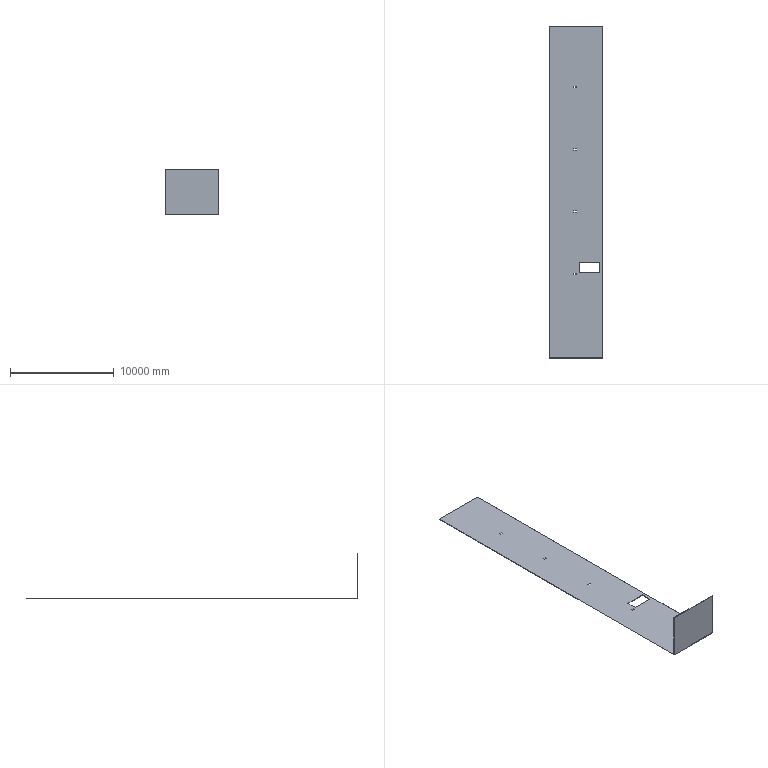Component | SolidWorks | ColorSteelTile-1 | 1 solid | 28 faces | box 5200 x 32004.68 x 4390.02 mm | volume 9342579455 mm3 | plane 28
build123d program:
from build123d import *

# Parameters (mm, degrees)
BOSS_EXTRUDE1_DEPTH       = 5200
CUT_EXTRUDE1_2_DEPTH      = 36550.396
CUT_EXTRUDE1_2_DEPTH_BACK = 36550.396
SKETCH2_W                 = 1000
SKETCH2_H                 = 2000.43
CUT_EXTRUDE1_DEPTH        = 36564.156
CUT_EXTRUDE1_DEPTH_BACK   = 36564.156
SKETCH1_W                 = 135
SKETCH1_H                 = 260


with BuildPart() as part:
    # Sketch1_2 → Boss-Extrude1 (new body)
    with BuildSketch(Plane.XY):
        Polygon((-3905.572, 113.12), (-35910.251, 113.12), (-35910.251, 4503.137), (-35860.251, 4503.137), (-35860.251, 163.12), (-3905.572, 163.12), align=None)
    extrude(amount=BOSS_EXTRUDE1_DEPTH)

    # Sketch2 → Cut-Extrude1_2 (cut, two sides: drawn at the far end of the back side and taken through both)
    with BuildSketch(Plane.XZ.offset(-113.12).offset(-CUT_EXTRUDE1_2_DEPTH_BACK)):
        with Locations((-27185.572, 3893.179)):
            Rectangle(SKETCH2_W, SKETCH2_H)
    extrude(amount=CUT_EXTRUDE1_2_DEPTH + CUT_EXTRUDE1_2_DEPTH_BACK, mode=Mode.SUBTRACT)

    # Sketch1 → Cut-Extrude1 (cut, two sides: drawn at the far end of the back side and taken through both)
    with BuildSketch(Plane(origin=(0, 0, 0), x_dir=(1, 0, 0), z_dir=(0, 1, 0)).offset(-CUT_EXTRUDE1_DEPTH_BACK)):
        with Locations((-9795.572, -2525)):
            Rectangle(SKETCH1_W, SKETCH1_H)
        with Locations((-15795.572, -2525)):
            Rectangle(SKETCH1_W, SKETCH1_H)
        with Locations((-21795.572, -2525)):
            Rectangle(SKETCH1_W, SKETCH1_H)
        with Locations((-27795.572, -2525)):
            Rectangle(SKETCH1_W, SKETCH1_H)
    extrude(amount=CUT_EXTRUDE1_DEPTH + CUT_EXTRUDE1_DEPTH_BACK, mode=Mode.SUBTRACT)


solid = part.part

# Placed as in the assembly
solid = solid.moved(Location((-830.074, 4663.226, -160.714), (90, 90, 0)))
STEP:
#1=CARTESIAN_POINT('',(61.611,-440.939,0.09473));
#2=VERTEX_POINT('',#1);
#3=CARTESIAN_POINT('',(71.847,-440.939,0.09473));
#4=VERTEX_POINT('',#3);
#5=CARTESIAN_POINT('',(1443.87,-440.939,0.09473));
#6=DIRECTION('',(1.,-0.,-0.));
#7=VECTOR('',#6,39.37);
#8=LINE('',#5,#7);
#9=EDGE_CURVE('',#2,#4,#8,.T.);
#10=ORIENTED_EDGE('',*,*,#9,.F.);
#11=CARTESIAN_POINT('',(61.611,-435.624,0.09473));
#12=VERTEX_POINT('',#11);
#13=CARTESIAN_POINT('',(61.611,29.829,0.09473));
#14=DIRECTION('',(-0.,-1.,0.));
#15=VECTOR('',#14,39.37);
#16=LINE('',#13,#15);
#17=EDGE_CURVE('',#12,#2,#16,.T.);
#18=ORIENTED_EDGE('',*,*,#17,.F.);
#19=CARTESIAN_POINT('',(71.847,-435.624,0.09473));
#20=VERTEX_POINT('',#19);
#21=CARTESIAN_POINT('',(1443.87,-435.624,0.09473));
#22=DIRECTION('',(-1.,0.,0.));
#23=VECTOR('',#22,39.37);
#24=LINE('',#21,#23);
#25=EDGE_CURVE('',#20,#12,#24,.T.);
#26=ORIENTED_EDGE('',*,*,#25,.F.);
#27=CARTESIAN_POINT('',(71.847,29.829,0.09473));
#28=DIRECTION('',(0.,1.,-0.));
#29=VECTOR('',#28,39.37);
#30=LINE('',#27,#29);
#31=EDGE_CURVE('',#4,#20,#30,.T.);
#32=ORIENTED_EDGE('',*,*,#31,.F.);
#33=EDGE_LOOP('',(#10,#18,#26,#32));
#34=FACE_BOUND('',#33,.T.);
#35=CARTESIAN_POINT('',(61.611,-913.38,0.09473));
#36=VERTEX_POINT('',#35);
#37=CARTESIAN_POINT('',(71.847,-913.38,0.09473));
#38=VERTEX_POINT('',#37);
#39=CARTESIAN_POINT('',(1443.87,-913.38,0.09473));
#40=DIRECTION('',(1.,-0.,-0.));
#41=VECTOR('',#40,39.37);
#42=LINE('',#39,#41);
#43=EDGE_CURVE('',#36,#38,#42,.T.);
#44=ORIENTED_EDGE('',*,*,#43,.F.);
#45=CARTESIAN_POINT('',(61.611,-908.065,0.09473));
#46=VERTEX_POINT('',#45);
#47=CARTESIAN_POINT('',(61.611,29.829,0.09473));
#48=DIRECTION('',(-0.,-1.,0.));
#49=VECTOR('',#48,39.37);
#50=LINE('',#47,#49);
#51=EDGE_CURVE('',#46,#36,#50,.T.);
#52=ORIENTED_EDGE('',*,*,#51,.F.);
#53=CARTESIAN_POINT('',(71.847,-908.065,0.09473));
#54=VERTEX_POINT('',#53);
#55=CARTESIAN_POINT('',(1443.87,-908.065,0.09473));
#56=DIRECTION('',(-1.,0.,0.));
#57=VECTOR('',#56,39.37);
#58=LINE('',#55,#57);
#59=EDGE_CURVE('',#54,#46,#58,.T.);
#60=ORIENTED_EDGE('',*,*,#59,.F.);
#61=CARTESIAN_POINT('',(71.847,29.829,0.09473));
#62=DIRECTION('',(0.,1.,-0.));
#63=VECTOR('',#62,39.37);
#64=LINE('',#61,#63);
#65=EDGE_CURVE('',#38,#54,#64,.T.);
#66=ORIENTED_EDGE('',*,*,#65,.F.);
#67=EDGE_LOOP('',(#44,#52,#60,#66));
#68=FACE_BOUND('',#67,.T.);
#69=CARTESIAN_POINT('',(159.973,-867.022,0.09473));
#70=VERTEX_POINT('',#69);
#71=CARTESIAN_POINT('',(159.973,-906.392,0.09473));
#72=VERTEX_POINT('',#71);
#73=CARTESIAN_POINT('',(159.973,29.829,0.09473));
#74=DIRECTION('',(0.,-1.,0.));
#75=VECTOR('',#74,39.37);
#76=LINE('',#73,#75);
#77=EDGE_CURVE('',#70,#72,#76,.T.);
#78=ORIENTED_EDGE('',*,*,#77,.T.);
#79=CARTESIAN_POINT('',(81.216,-906.392,0.09473));
#80=VERTEX_POINT('',#79);
#81=CARTESIAN_POINT('',(1443.87,-906.392,0.09473));
#82=DIRECTION('',(-1.,0.,0.));
#83=VECTOR('',#82,39.37);
#84=LINE('',#81,#83);
#85=EDGE_CURVE('',#72,#80,#84,.T.);
#86=ORIENTED_EDGE('',*,*,#85,.T.);
#87=CARTESIAN_POINT('',(81.216,-867.022,0.09473));
#88=VERTEX_POINT('',#87);
#89=CARTESIAN_POINT('',(81.216,29.829,0.09473));
#90=DIRECTION('',(0.,1.,-0.));
#91=VECTOR('',#90,39.37);
#92=LINE('',#89,#91);
#93=EDGE_CURVE('',#80,#88,#92,.T.);
#94=ORIENTED_EDGE('',*,*,#93,.T.);
#95=CARTESIAN_POINT('',(1443.87,-867.022,0.09473));
#96=DIRECTION('',(1.,-0.,-0.));
#97=VECTOR('',#96,39.37);
#98=LINE('',#95,#97);
#99=EDGE_CURVE('',#88,#70,#98,.T.);
#100=ORIENTED_EDGE('',*,*,#99,.T.);
#101=EDGE_LOOP('',(#78,#86,#94,#100));
#102=FACE_BOUND('',#101,.T.);
#103=CARTESIAN_POINT('',(172.044,29.829,0.09473));
#104=VERTEX_POINT('',#103);
#105=CARTESIAN_POINT('',(172.044,-1228.229,0.09473));
#106=VERTEX_POINT('',#105);
#107=CARTESIAN_POINT('',(172.044,29.829,0.09473));
#108=DIRECTION('',(0.,-1.,0.));
#109=VECTOR('',#108,39.37);
#110=LINE('',#107,#109);
#111=EDGE_CURVE('',#104,#106,#110,.T.);
#112=ORIENTED_EDGE('',*,*,#111,.F.);
#113=CARTESIAN_POINT('',(-32.68,29.829,0.09473));
#114=VERTEX_POINT('',#113);
#115=CARTESIAN_POINT('',(1443.87,29.829,0.09473));
#116=DIRECTION('',(-1.,0.,0.));
#117=VECTOR('',#116,39.37);
#118=LINE('',#115,#117);
#119=EDGE_CURVE('',#104,#114,#118,.T.);
#120=ORIENTED_EDGE('',*,*,#119,.T.);
#121=CARTESIAN_POINT('',(-32.68,-1228.229,0.09473));
#122=VERTEX_POINT('',#121);
#123=CARTESIAN_POINT('',(-32.68,29.829,0.09473));
#124=DIRECTION('',(-0.,-1.,0.));
#125=VECTOR('',#124,39.37);
#126=LINE('',#123,#125);
#127=EDGE_CURVE('',#114,#122,#126,.T.);
#128=ORIENTED_EDGE('',*,*,#127,.T.);
#129=CARTESIAN_POINT('',(1443.87,-1228.229,0.09473));
#130=DIRECTION('',(-1.,0.,0.));
#131=VECTOR('',#130,39.37);
#132=LINE('',#129,#131);
#133=EDGE_CURVE('',#106,#122,#132,.T.);
#134=ORIENTED_EDGE('',*,*,#133,.F.);
#135=EDGE_LOOP('',(#112,#120,#128,#134));
#136=FACE_OUTER_BOUND('',#135,.T.);
#137=CARTESIAN_POINT('',(61.611,-677.159,0.09473));
#138=VERTEX_POINT('',#137);
#139=CARTESIAN_POINT('',(71.847,-677.159,0.09473));
#140=VERTEX_POINT('',#139);
#141=CARTESIAN_POINT('',(1443.87,-677.159,0.09473));
#142=DIRECTION('',(1.,-0.,-0.));
#143=VECTOR('',#142,39.37);
#144=LINE('',#141,#143);
#145=EDGE_CURVE('',#138,#140,#144,.T.);
#146=ORIENTED_EDGE('',*,*,#145,.F.);
#147=CARTESIAN_POINT('',(61.611,-671.844,0.09473));
#148=VERTEX_POINT('',#147);
#149=CARTESIAN_POINT('',(61.611,29.829,0.09473));
#150=DIRECTION('',(-0.,-1.,0.));
#151=VECTOR('',#150,39.37);
#152=LINE('',#149,#151);
#153=EDGE_CURVE('',#148,#138,#152,.T.);
#154=ORIENTED_EDGE('',*,*,#153,.F.);
#155=CARTESIAN_POINT('',(71.847,-671.844,0.09473));
#156=VERTEX_POINT('',#155);
#157=CARTESIAN_POINT('',(1443.87,-671.844,0.09473));
#158=DIRECTION('',(-1.,0.,0.));
#159=VECTOR('',#158,39.37);
#160=LINE('',#157,#159);
#161=EDGE_CURVE('',#156,#148,#160,.T.);
#162=ORIENTED_EDGE('',*,*,#161,.F.);
#163=CARTESIAN_POINT('',(71.847,29.829,0.09473));
#164=DIRECTION('',(0.,1.,-0.));
#165=VECTOR('',#164,39.37);
#166=LINE('',#163,#165);
#167=EDGE_CURVE('',#140,#156,#166,.T.);
#168=ORIENTED_EDGE('',*,*,#167,.F.);
#169=EDGE_LOOP('',(#146,#154,#162,#168));
#170=FACE_BOUND('',#169,.T.);
#171=CARTESIAN_POINT('',(61.611,-204.718,0.09473));
#172=VERTEX_POINT('',#171);
#173=CARTESIAN_POINT('',(71.847,-204.718,0.09473));
#174=VERTEX_POINT('',#173);
#175=CARTESIAN_POINT('',(1443.87,-204.718,0.09473));
#176=DIRECTION('',(1.,-0.,-0.));
#177=VECTOR('',#176,39.37);
#178=LINE('',#175,#177);
#179=EDGE_CURVE('',#172,#174,#178,.T.);
#180=ORIENTED_EDGE('',*,*,#179,.F.);
#181=CARTESIAN_POINT('',(61.611,-199.403,0.09473));
#182=VERTEX_POINT('',#181);
#183=CARTESIAN_POINT('',(61.611,29.829,0.09473));
#184=DIRECTION('',(-0.,-1.,0.));
#185=VECTOR('',#184,39.37);
#186=LINE('',#183,#185);
#187=EDGE_CURVE('',#182,#172,#186,.T.);
#188=ORIENTED_EDGE('',*,*,#187,.F.);
#189=CARTESIAN_POINT('',(71.847,-199.403,0.09473));
#190=VERTEX_POINT('',#189);
#191=CARTESIAN_POINT('',(1443.87,-199.403,0.09473));
#192=DIRECTION('',(-1.,0.,0.));
#193=VECTOR('',#192,39.37);
#194=LINE('',#191,#193);
#195=EDGE_CURVE('',#190,#182,#194,.T.);
#196=ORIENTED_EDGE('',*,*,#195,.F.);
#197=CARTESIAN_POINT('',(71.847,29.829,0.09473));
#198=DIRECTION('',(0.,1.,-0.));
#199=VECTOR('',#198,39.37);
#200=LINE('',#197,#199);
#201=EDGE_CURVE('',#174,#190,#200,.T.);
#202=ORIENTED_EDGE('',*,*,#201,.F.);
#203=EDGE_LOOP('',(#180,#188,#196,#202));
#204=FACE_BOUND('',#203,.T.);
#205=CARTESIAN_POINT('',(1443.87,29.829,0.09473));
#206=DIRECTION('',(-0.,-0.,-1.));
#207=DIRECTION('',(-1.,0.,0.));
#208=AXIS2_PLACEMENT_3D('',#205,#206,#207);
#209=PLANE('',#208);
#210=ADVANCED_FACE('',(#34,#68,#102,#136,#170,#204),#209,.F.);
#211=CARTESIAN_POINT('',(71.847,-440.939,-1.874));
#212=VERTEX_POINT('',#211);
#213=CARTESIAN_POINT('',(61.611,-440.939,-1.874));
#214=VERTEX_POINT('',#213);
#215=CARTESIAN_POINT('',(1443.87,-440.939,-1.874));
#216=DIRECTION('',(-1.,0.,0.));
#217=VECTOR('',#216,39.37);
#218=LINE('',#215,#217);
#219=EDGE_CURVE('',#212,#214,#218,.T.);
#220=ORIENTED_EDGE('',*,*,#219,.F.);
#221=CARTESIAN_POINT('',(71.847,-435.624,-1.874));
#222=VERTEX_POINT('',#221);
#223=CARTESIAN_POINT('',(71.847,29.829,-1.874));
#224=DIRECTION('',(-0.,-1.,0.));
#225=VECTOR('',#224,39.37);
#226=LINE('',#223,#225);
#227=EDGE_CURVE('',#222,#212,#226,.T.);
#228=ORIENTED_EDGE('',*,*,#227,.F.);
#229=CARTESIAN_POINT('',(61.611,-435.624,-1.874));
#230=VERTEX_POINT('',#229);
#231=CARTESIAN_POINT('',(1443.87,-435.624,-1.874));
#232=DIRECTION('',(1.,-0.,-0.));
#233=VECTOR('',#232,39.37);
#234=LINE('',#231,#233);
#235=EDGE_CURVE('',#230,#222,#234,.T.);
#236=ORIENTED_EDGE('',*,*,#235,.F.);
#237=CARTESIAN_POINT('',(61.611,29.829,-1.874));
#238=DIRECTION('',(0.,1.,-0.));
#239=VECTOR('',#238,39.37);
#240=LINE('',#237,#239);
#241=EDGE_CURVE('',#214,#230,#240,.T.);
#242=ORIENTED_EDGE('',*,*,#241,.F.);
#243=EDGE_LOOP('',(#220,#228,#236,#242));
#244=FACE_BOUND('',#243,.T.);
#245=CARTESIAN_POINT('',(71.847,-913.38,-1.874));
#246=VERTEX_POINT('',#245);
#247=CARTESIAN_POINT('',(61.611,-913.38,-1.874));
#248=VERTEX_POINT('',#247);
#249=CARTESIAN_POINT('',(1443.87,-913.38,-1.874));
#250=DIRECTION('',(-1.,0.,0.));
#251=VECTOR('',#250,39.37);
#252=LINE('',#249,#251);
#253=EDGE_CURVE('',#246,#248,#252,.T.);
#254=ORIENTED_EDGE('',*,*,#253,.F.);
#255=CARTESIAN_POINT('',(71.847,-908.065,-1.874));
#256=VERTEX_POINT('',#255);
#257=CARTESIAN_POINT('',(71.847,29.829,-1.874));
#258=DIRECTION('',(-0.,-1.,0.));
#259=VECTOR('',#258,39.37);
#260=LINE('',#257,#259);
#261=EDGE_CURVE('',#256,#246,#260,.T.);
#262=ORIENTED_EDGE('',*,*,#261,.F.);
#263=CARTESIAN_POINT('',(61.611,-908.065,-1.874));
#264=VERTEX_POINT('',#263);
#265=CARTESIAN_POINT('',(1443.87,-908.065,-1.874));
#266=DIRECTION('',(1.,-0.,-0.));
#267=VECTOR('',#266,39.37);
#268=LINE('',#265,#267);
#269=EDGE_CURVE('',#264,#256,#268,.T.);
#270=ORIENTED_EDGE('',*,*,#269,.F.);
#271=CARTESIAN_POINT('',(61.611,29.829,-1.874));
#272=DIRECTION('',(0.,1.,-0.));
#273=VECTOR('',#272,39.37);
#274=LINE('',#271,#273);
#275=EDGE_CURVE('',#248,#264,#274,.T.);
#276=ORIENTED_EDGE('',*,*,#275,.F.);
#277=EDGE_LOOP('',(#254,#262,#270,#276));
#278=FACE_BOUND('',#277,.T.);
#279=CARTESIAN_POINT('',(81.216,-867.022,-1.874));
#280=VERTEX_POINT('',#279);
#281=CARTESIAN_POINT('',(81.216,-906.392,-1.874));
#282=VERTEX_POINT('',#281);
#283=CARTESIAN_POINT('',(81.216,29.829,-1.874));
#284=DIRECTION('',(-0.,-1.,0.));
#285=VECTOR('',#284,39.37);
#286=LINE('',#283,#285);
#287=EDGE_CURVE('',#280,#282,#286,.T.);
#288=ORIENTED_EDGE('',*,*,#287,.T.);
#289=CARTESIAN_POINT('',(159.973,-906.392,-1.874));
#290=VERTEX_POINT('',#289);
#291=CARTESIAN_POINT('',(1443.87,-906.392,-1.874));
#292=DIRECTION('',(1.,-0.,-0.));
#293=VECTOR('',#292,39.37);
#294=LINE('',#291,#293);
#295=EDGE_CURVE('',#282,#290,#294,.T.);
#296=ORIENTED_EDGE('',*,*,#295,.T.);
#297=CARTESIAN_POINT('',(159.973,-867.022,-1.874));
#298=VERTEX_POINT('',#297);
#299=CARTESIAN_POINT('',(159.973,29.829,-1.874));
#300=DIRECTION('',(-0.,1.,-0.));
#301=VECTOR('',#300,39.37);
#302=LINE('',#299,#301);
#303=EDGE_CURVE('',#290,#298,#302,.T.);
#304=ORIENTED_EDGE('',*,*,#303,.T.);
#305=CARTESIAN_POINT('',(1443.87,-867.022,-1.874));
#306=DIRECTION('',(-1.,0.,0.));
#307=VECTOR('',#306,39.37);
#308=LINE('',#305,#307);
#309=EDGE_CURVE('',#298,#280,#308,.T.);
#310=ORIENTED_EDGE('',*,*,#309,.T.);
#311=EDGE_LOOP('',(#288,#296,#304,#310));
#312=FACE_BOUND('',#311,.T.);
#313=CARTESIAN_POINT('',(172.044,-1230.198,-1.874));
#314=VERTEX_POINT('',#313);
#315=CARTESIAN_POINT('',(172.044,29.829,-1.874));
#316=VERTEX_POINT('',#315);
#317=CARTESIAN_POINT('',(172.044,29.829,-1.874));
#318=DIRECTION('',(0.,1.,-0.));
#319=VECTOR('',#318,39.37);
#320=LINE('',#317,#319);
#321=EDGE_CURVE('',#314,#316,#320,.T.);
#322=ORIENTED_EDGE('',*,*,#321,.F.);
#323=CARTESIAN_POINT('',(-32.68,-1230.198,-1.874));
#324=VERTEX_POINT('',#323);
#325=CARTESIAN_POINT('',(1443.87,-1230.198,-1.874));
#326=DIRECTION('',(-1.,0.,0.));
#327=VECTOR('',#326,39.37);
#328=LINE('',#325,#327);
#329=EDGE_CURVE('',#314,#324,#328,.T.);
#330=ORIENTED_EDGE('',*,*,#329,.T.);
#331=CARTESIAN_POINT('',(-32.68,29.829,-1.874));
#332=VERTEX_POINT('',#331);
#333=CARTESIAN_POINT('',(-32.68,29.829,-1.874));
#334=DIRECTION('',(0.,1.,-0.));
#335=VECTOR('',#334,39.37);
#336=LINE('',#333,#335);
#337=EDGE_CURVE('',#324,#332,#336,.T.);
#338=ORIENTED_EDGE('',*,*,#337,.T.);
#339=CARTESIAN_POINT('',(1443.87,29.829,-1.874));
#340=DIRECTION('',(-1.,0.,0.));
#341=VECTOR('',#340,39.37);
#342=LINE('',#339,#341);
#343=EDGE_CURVE('',#316,#332,#342,.T.);
#344=ORIENTED_EDGE('',*,*,#343,.F.);
#345=EDGE_LOOP('',(#322,#330,#338,#344));
#346=FACE_OUTER_BOUND('',#345,.T.);
#347=CARTESIAN_POINT('',(71.847,-677.159,-1.874));
#348=VERTEX_POINT('',#347);
#349=CARTESIAN_POINT('',(61.611,-677.159,-1.874));
#350=VERTEX_POINT('',#349);
#351=CARTESIAN_POINT('',(1443.87,-677.159,-1.874));
#352=DIRECTION('',(-1.,0.,0.));
#353=VECTOR('',#352,39.37);
#354=LINE('',#351,#353);
#355=EDGE_CURVE('',#348,#350,#354,.T.);
#356=ORIENTED_EDGE('',*,*,#355,.F.);
#357=CARTESIAN_POINT('',(71.847,-671.844,-1.874));
#358=VERTEX_POINT('',#357);
#359=CARTESIAN_POINT('',(71.847,29.829,-1.874));
#360=DIRECTION('',(-0.,-1.,0.));
#361=VECTOR('',#360,39.37);
#362=LINE('',#359,#361);
#363=EDGE_CURVE('',#358,#348,#362,.T.);
#364=ORIENTED_EDGE('',*,*,#363,.F.);
#365=CARTESIAN_POINT('',(61.611,-671.844,-1.874));
#366=VERTEX_POINT('',#365);
#367=CARTESIAN_POINT('',(1443.87,-671.844,-1.874));
#368=DIRECTION('',(1.,-0.,-0.));
#369=VECTOR('',#368,39.37);
#370=LINE('',#367,#369);
#371=EDGE_CURVE('',#366,#358,#370,.T.);
#372=ORIENTED_EDGE('',*,*,#371,.F.);
#373=CARTESIAN_POINT('',(61.611,29.829,-1.874));
#374=DIRECTION('',(0.,1.,-0.));
#375=VECTOR('',#374,39.37);
#376=LINE('',#373,#375);
#377=EDGE_CURVE('',#350,#366,#376,.T.);
#378=ORIENTED_EDGE('',*,*,#377,.F.);
#379=EDGE_LOOP('',(#356,#364,#372,#378));
#380=FACE_BOUND('',#379,.T.);
#381=CARTESIAN_POINT('',(71.847,-204.718,-1.874));
#382=VERTEX_POINT('',#381);
#383=CARTESIAN_POINT('',(61.611,-204.718,-1.874));
#384=VERTEX_POINT('',#383);
#385=CARTESIAN_POINT('',(1443.87,-204.718,-1.874));
#386=DIRECTION('',(-1.,0.,0.));
#387=VECTOR('',#386,39.37);
#388=LINE('',#385,#387);
#389=EDGE_CURVE('',#382,#384,#388,.T.);
#390=ORIENTED_EDGE('',*,*,#389,.F.);
#391=CARTESIAN_POINT('',(71.847,-199.403,-1.874));
#392=VERTEX_POINT('',#391);
#393=CARTESIAN_POINT('',(71.847,29.829,-1.874));
#394=DIRECTION('',(-0.,-1.,0.));
#395=VECTOR('',#394,39.37);
#396=LINE('',#393,#395);
#397=EDGE_CURVE('',#392,#382,#396,.T.);
#398=ORIENTED_EDGE('',*,*,#397,.F.);
#399=CARTESIAN_POINT('',(61.611,-199.403,-1.874));
#400=VERTEX_POINT('',#399);
#401=CARTESIAN_POINT('',(1443.87,-199.403,-1.874));
#402=DIRECTION('',(1.,-0.,-0.));
#403=VECTOR('',#402,39.37);
#404=LINE('',#401,#403);
#405=EDGE_CURVE('',#400,#392,#404,.T.);
#406=ORIENTED_EDGE('',*,*,#405,.F.);
#407=CARTESIAN_POINT('',(61.611,29.829,-1.874));
#408=DIRECTION('',(0.,1.,-0.));
#409=VECTOR('',#408,39.37);
#410=LINE('',#407,#409);
#411=EDGE_CURVE('',#384,#400,#410,.T.);
#412=ORIENTED_EDGE('',*,*,#411,.F.);
#413=EDGE_LOOP('',(#390,#398,#406,#412));
#414=FACE_BOUND('',#413,.T.);
#415=CARTESIAN_POINT('',(1443.87,29.829,-1.874));
#416=DIRECTION('',(0.,0.,1.));
#417=DIRECTION('',(1.,-0.,-0.));
#418=AXIS2_PLACEMENT_3D('',#415,#416,#417);
#419=PLANE('',#418);
#420=ADVANCED_FACE('',(#244,#278,#312,#346,#380,#414),#419,.F.);
#421=CARTESIAN_POINT('',(172.044,29.829,-1.874));
#422=DIRECTION('',(0.,0.,1.));
#423=VECTOR('',#422,39.37);
#424=LINE('',#421,#423);
#425=EDGE_CURVE('',#316,#104,#424,.T.);
#426=ORIENTED_EDGE('',*,*,#425,.F.);
#427=ORIENTED_EDGE('',*,*,#343,.T.);
#428=CARTESIAN_POINT('',(-32.68,29.829,-1.874));
#429=DIRECTION('',(0.,0.,1.));
#430=VECTOR('',#429,39.37);
#431=LINE('',#428,#430);
#432=EDGE_CURVE('',#332,#114,#431,.T.);
#433=ORIENTED_EDGE('',*,*,#432,.T.);
#434=ORIENTED_EDGE('',*,*,#119,.F.);
#435=EDGE_LOOP('',(#426,#427,#433,#434));
#436=FACE_OUTER_BOUND('',#435,.T.);
#437=CARTESIAN_POINT('',(1443.87,29.829,-1.874));
#438=DIRECTION('',(-0.,-1.,0.));
#439=DIRECTION('',(1.,-0.,-0.));
#440=AXIS2_PLACEMENT_3D('',#437,#438,#439);
#441=PLANE('',#440);
#442=ADVANCED_FACE('',(#436),#441,.F.);
#443=CARTESIAN_POINT('',(172.044,-1228.229,170.962));
#444=VERTEX_POINT('',#443);
#445=CARTESIAN_POINT('',(172.044,-1228.229,0.09473));
#446=DIRECTION('',(0.,0.,1.));
#447=VECTOR('',#446,39.37);
#448=LINE('',#445,#447);
#449=EDGE_CURVE('',#106,#444,#448,.T.);
#450=ORIENTED_EDGE('',*,*,#449,.F.);
#451=ORIENTED_EDGE('',*,*,#133,.T.);
#452=CARTESIAN_POINT('',(-32.68,-1228.229,170.962));
#453=VERTEX_POINT('',#452);
#454=CARTESIAN_POINT('',(-32.68,-1228.229,0.09473));
#455=DIRECTION('',(0.,0.,1.));
#456=VECTOR('',#455,39.37);
#457=LINE('',#454,#456);
#458=EDGE_CURVE('',#122,#453,#457,.T.);
#459=ORIENTED_EDGE('',*,*,#458,.T.);
#460=CARTESIAN_POINT('',(1443.87,-1228.229,170.962));
#461=DIRECTION('',(-1.,0.,0.));
#462=VECTOR('',#461,39.37);
#463=LINE('',#460,#462);
#464=EDGE_CURVE('',#444,#453,#463,.T.);
#465=ORIENTED_EDGE('',*,*,#464,.F.);
#466=EDGE_LOOP('',(#450,#451,#459,#465));
#467=FACE_OUTER_BOUND('',#466,.T.);
#468=CARTESIAN_POINT('',(1443.87,-1228.229,0.09473));
#469=DIRECTION('',(-0.,-1.,0.));
#470=DIRECTION('',(1.,-0.,-0.));
#471=AXIS2_PLACEMENT_3D('',#468,#469,#470);
#472=PLANE('',#471);
#473=ADVANCED_FACE('',(#467),#472,.F.);
#474=CARTESIAN_POINT('',(172.044,-1230.198,170.962));
#475=VERTEX_POINT('',#474);
#476=CARTESIAN_POINT('',(172.044,-1228.229,170.962));
#477=DIRECTION('',(0.,-1.,0.));
#478=VECTOR('',#477,39.37);
#479=LINE('',#476,#478);
#480=EDGE_CURVE('',#444,#475,#479,.T.);
#481=ORIENTED_EDGE('',*,*,#480,.F.);
#482=ORIENTED_EDGE('',*,*,#464,.T.);
#483=CARTESIAN_POINT('',(-32.68,-1230.198,170.962));
#484=VERTEX_POINT('',#483);
#485=CARTESIAN_POINT('',(-32.68,-1228.229,170.962));
#486=DIRECTION('',(-0.,-1.,0.));
#487=VECTOR('',#486,39.37);
#488=LINE('',#485,#487);
#489=EDGE_CURVE('',#453,#484,#488,.T.);
#490=ORIENTED_EDGE('',*,*,#489,.T.);
#491=CARTESIAN_POINT('',(1443.87,-1230.198,170.962));
#492=DIRECTION('',(-1.,0.,0.));
#493=VECTOR('',#492,39.37);
#494=LINE('',#491,#493);
#495=EDGE_CURVE('',#475,#484,#494,.T.);
#496=ORIENTED_EDGE('',*,*,#495,.F.);
#497=EDGE_LOOP('',(#481,#482,#490,#496));
#498=FACE_OUTER_BOUND('',#497,.T.);
#499=CARTESIAN_POINT('',(1443.87,-1228.229,170.962));
#500=DIRECTION('',(-0.,-0.,-1.));
#501=DIRECTION('',(-1.,0.,0.));
#502=AXIS2_PLACEMENT_3D('',#499,#500,#501);
#503=PLANE('',#502);
#504=ADVANCED_FACE('',(#498),#503,.F.);
#505=CARTESIAN_POINT('',(172.044,-1230.198,-1.874));
#506=DIRECTION('',(0.,-0.,-1.));
#507=VECTOR('',#506,39.37);
#508=LINE('',#505,#507);
#509=EDGE_CURVE('',#475,#314,#508,.T.);
#510=ORIENTED_EDGE('',*,*,#509,.F.);
#511=ORIENTED_EDGE('',*,*,#495,.T.);
#512=CARTESIAN_POINT('',(-32.68,-1230.198,-1.874));
#513=DIRECTION('',(-0.,-0.,-1.));
#514=VECTOR('',#513,39.37);
#515=LINE('',#512,#514);
#516=EDGE_CURVE('',#484,#324,#515,.T.);
#517=ORIENTED_EDGE('',*,*,#516,.T.);
#518=ORIENTED_EDGE('',*,*,#329,.F.);
#519=EDGE_LOOP('',(#510,#511,#517,#518));
#520=FACE_OUTER_BOUND('',#519,.T.);
#521=CARTESIAN_POINT('',(1443.87,-1230.198,-1.874));
#522=DIRECTION('',(0.,1.,-0.));
#523=DIRECTION('',(-1.,0.,0.));
#524=AXIS2_PLACEMENT_3D('',#521,#522,#523);
#525=PLANE('',#524);
#526=ADVANCED_FACE('',(#520),#525,.F.);
#527=ORIENTED_EDGE('',*,*,#432,.F.);
#528=ORIENTED_EDGE('',*,*,#337,.F.);
#529=ORIENTED_EDGE('',*,*,#516,.F.);
#530=ORIENTED_EDGE('',*,*,#489,.F.);
#531=ORIENTED_EDGE('',*,*,#458,.F.);
#532=ORIENTED_EDGE('',*,*,#127,.F.);
#533=EDGE_LOOP('',(#527,#528,#529,#530,#531,#532));
#534=FACE_OUTER_BOUND('',#533,.T.);
#535=CARTESIAN_POINT('',(-32.68,183.592,-6.327));
#536=DIRECTION('',(1.,-0.,-0.));
#537=DIRECTION('',(0.,1.,-0.));
#538=AXIS2_PLACEMENT_3D('',#535,#536,#537);
#539=PLANE('',#538);
#540=ADVANCED_FACE('',(#534),#539,.F.);
#541=ORIENTED_EDGE('',*,*,#321,.T.);
#542=ORIENTED_EDGE('',*,*,#425,.T.);
#543=ORIENTED_EDGE('',*,*,#111,.T.);
#544=ORIENTED_EDGE('',*,*,#449,.T.);
#545=ORIENTED_EDGE('',*,*,#480,.T.);
#546=ORIENTED_EDGE('',*,*,#509,.T.);
#547=EDGE_LOOP('',(#541,#542,#543,#544,#545,#546));
#548=FACE_OUTER_BOUND('',#547,.T.);
#549=CARTESIAN_POINT('',(172.044,-705.073,-17.704));
#550=DIRECTION('',(1.,0.,-0.));
#551=DIRECTION('',(0.,-0.,-1.));
#552=AXIS2_PLACEMENT_3D('',#549,#550,#551);
#553=PLANE('',#552);
#554=ADVANCED_FACE('',(#548),#553,.T.);
#555=CARTESIAN_POINT('',(159.973,-906.392,170.962));
#556=DIRECTION('',(-0.,0.,-1.));
#557=VECTOR('',#556,39.37);
#558=LINE('',#555,#557);
#559=EDGE_CURVE('',#72,#290,#558,.T.);
#560=ORIENTED_EDGE('',*,*,#559,.T.);
#561=ORIENTED_EDGE('',*,*,#295,.F.);
#562=CARTESIAN_POINT('',(81.216,-906.392,170.962));
#563=DIRECTION('',(-0.,0.,-1.));
#564=VECTOR('',#563,39.37);
#565=LINE('',#562,#564);
#566=EDGE_CURVE('',#80,#282,#565,.T.);
#567=ORIENTED_EDGE('',*,*,#566,.F.);
#568=ORIENTED_EDGE('',*,*,#85,.F.);
#569=EDGE_LOOP('',(#560,#561,#567,#568));
#570=FACE_OUTER_BOUND('',#569,.T.);
#571=CARTESIAN_POINT('',(159.973,-906.392,170.962));
#572=DIRECTION('',(-0.,-1.,-0.));
#573=DIRECTION('',(-0.,0.,-1.));
#574=AXIS2_PLACEMENT_3D('',#571,#572,#573);
#575=PLANE('',#574);
#576=ADVANCED_FACE('',(#570),#575,.F.);
#577=CARTESIAN_POINT('',(159.973,-867.022,170.962));
#578=DIRECTION('',(-0.,0.,-1.));
#579=VECTOR('',#578,39.37);
#580=LINE('',#577,#579);
#581=EDGE_CURVE('',#70,#298,#580,.T.);
#582=ORIENTED_EDGE('',*,*,#581,.T.);
#583=ORIENTED_EDGE('',*,*,#303,.F.);
#584=ORIENTED_EDGE('',*,*,#559,.F.);
#585=ORIENTED_EDGE('',*,*,#77,.F.);
#586=EDGE_LOOP('',(#582,#583,#584,#585));
#587=FACE_OUTER_BOUND('',#586,.T.);
#588=CARTESIAN_POINT('',(159.973,-906.392,170.962));
#589=DIRECTION('',(1.,0.,-0.));
#590=DIRECTION('',(-0.,1.,-0.));
#591=AXIS2_PLACEMENT_3D('',#588,#589,#590);
#592=PLANE('',#591);
#593=ADVANCED_FACE('',(#587),#592,.F.);
#594=CARTESIAN_POINT('',(81.216,-867.022,170.962));
#595=DIRECTION('',(-0.,0.,-1.));
#596=VECTOR('',#595,39.37);
#597=LINE('',#594,#596);
#598=EDGE_CURVE('',#88,#280,#597,.T.);
#599=ORIENTED_EDGE('',*,*,#598,.T.);
#600=ORIENTED_EDGE('',*,*,#309,.F.);
#601=ORIENTED_EDGE('',*,*,#581,.F.);
#602=ORIENTED_EDGE('',*,*,#99,.F.);
#603=EDGE_LOOP('',(#599,#600,#601,#602));
#604=FACE_OUTER_BOUND('',#603,.T.);
#605=CARTESIAN_POINT('',(159.973,-867.022,170.962));
#606=DIRECTION('',(0.,1.,0.));
#607=DIRECTION('',(0.,-0.,1.));
#608=AXIS2_PLACEMENT_3D('',#605,#606,#607);
#609=PLANE('',#608);
#610=ADVANCED_FACE('',(#604),#609,.F.);
#611=ORIENTED_EDGE('',*,*,#566,.T.);
#612=ORIENTED_EDGE('',*,*,#287,.F.);
#613=ORIENTED_EDGE('',*,*,#598,.F.);
#614=ORIENTED_EDGE('',*,*,#93,.F.);
#615=EDGE_LOOP('',(#611,#612,#613,#614));
#616=FACE_OUTER_BOUND('',#615,.T.);
#617=CARTESIAN_POINT('',(81.216,-906.392,170.962));
#618=DIRECTION('',(-1.,0.,0.));
#619=DIRECTION('',(-0.,-1.,0.));
#620=AXIS2_PLACEMENT_3D('',#617,#618,#619);
#621=PLANE('',#620);
#622=ADVANCED_FACE('',(#616),#621,.F.);
#623=ORIENTED_EDGE('',*,*,#43,.T.);
#624=CARTESIAN_POINT('',(71.847,-913.38,-1.874));
#625=DIRECTION('',(-0.,-0.,-1.));
#626=VECTOR('',#625,39.37);
#627=LINE('',#624,#626);
#628=EDGE_CURVE('',#38,#246,#627,.T.);
#629=ORIENTED_EDGE('',*,*,#628,.T.);
#630=ORIENTED_EDGE('',*,*,#253,.T.);
#631=CARTESIAN_POINT('',(61.611,-913.38,-1.874));
#632=DIRECTION('',(-0.,-0.,-1.));
#633=VECTOR('',#632,39.37);
#634=LINE('',#631,#633);
#635=EDGE_CURVE('',#36,#248,#634,.T.);
#636=ORIENTED_EDGE('',*,*,#635,.F.);
#637=EDGE_LOOP('',(#623,#629,#630,#636));
#638=FACE_OUTER_BOUND('',#637,.T.);
#639=CARTESIAN_POINT('',(61.611,-913.38,-1.874));
#640=DIRECTION('',(0.,1.,-0.));
#641=DIRECTION('',(-1.,0.,0.));
#642=AXIS2_PLACEMENT_3D('',#639,#640,#641);
#643=PLANE('',#642);
#644=ADVANCED_FACE('',(#638),#643,.T.);
#645=ORIENTED_EDGE('',*,*,#65,.T.);
#646=CARTESIAN_POINT('',(71.847,-908.065,-1.874));
#647=DIRECTION('',(-0.,-0.,-1.));
#648=VECTOR('',#647,39.37);
#649=LINE('',#646,#648);
#650=EDGE_CURVE('',#54,#256,#649,.T.);
#651=ORIENTED_EDGE('',*,*,#650,.T.);
#652=ORIENTED_EDGE('',*,*,#261,.T.);
#653=ORIENTED_EDGE('',*,*,#628,.F.);
#654=EDGE_LOOP('',(#645,#651,#652,#653));
#655=FACE_OUTER_BOUND('',#654,.T.);
#656=CARTESIAN_POINT('',(71.847,-913.38,-1.874));
#657=DIRECTION('',(-1.,0.,0.));
#658=DIRECTION('',(-0.,-1.,0.));
#659=AXIS2_PLACEMENT_3D('',#656,#657,#658);
#660=PLANE('',#659);
#661=ADVANCED_FACE('',(#655),#660,.T.);
#662=ORIENTED_EDGE('',*,*,#59,.T.);
#663=CARTESIAN_POINT('',(61.611,-908.065,-1.874));
#664=DIRECTION('',(-0.,-0.,-1.));
#665=VECTOR('',#664,39.37);
#666=LINE('',#663,#665);
#667=EDGE_CURVE('',#46,#264,#666,.T.);
#668=ORIENTED_EDGE('',*,*,#667,.T.);
#669=ORIENTED_EDGE('',*,*,#269,.T.);
#670=ORIENTED_EDGE('',*,*,#650,.F.);
#671=EDGE_LOOP('',(#662,#668,#669,#670));
#672=FACE_OUTER_BOUND('',#671,.T.);
#673=CARTESIAN_POINT('',(61.611,-908.065,-1.874));
#674=DIRECTION('',(-0.,-1.,0.));
#675=DIRECTION('',(1.,-0.,-0.));
#676=AXIS2_PLACEMENT_3D('',#673,#674,#675);
#677=PLANE('',#676);
#678=ADVANCED_FACE('',(#672),#677,.T.);
#679=ORIENTED_EDGE('',*,*,#51,.T.);
#680=ORIENTED_EDGE('',*,*,#635,.T.);
#681=ORIENTED_EDGE('',*,*,#275,.T.);
#682=ORIENTED_EDGE('',*,*,#667,.F.);
#683=EDGE_LOOP('',(#679,#680,#681,#682));
#684=FACE_OUTER_BOUND('',#683,.T.);
#685=CARTESIAN_POINT('',(61.611,-913.38,-1.874));
#686=DIRECTION('',(1.,-0.,-0.));
#687=DIRECTION('',(0.,1.,-0.));
#688=AXIS2_PLACEMENT_3D('',#685,#686,#687);
#689=PLANE('',#688);
#690=ADVANCED_FACE('',(#684),#689,.T.);
#691=ORIENTED_EDGE('',*,*,#145,.T.);
#692=CARTESIAN_POINT('',(71.847,-677.159,-1.874));
#693=DIRECTION('',(-0.,-0.,-1.));
#694=VECTOR('',#693,39.37);
#695=LINE('',#692,#694);
#696=EDGE_CURVE('',#140,#348,#695,.T.);
#697=ORIENTED_EDGE('',*,*,#696,.T.);
#698=ORIENTED_EDGE('',*,*,#355,.T.);
#699=CARTESIAN_POINT('',(61.611,-677.159,-1.874));
#700=DIRECTION('',(-0.,-0.,-1.));
#701=VECTOR('',#700,39.37);
#702=LINE('',#699,#701);
#703=EDGE_CURVE('',#138,#350,#702,.T.);
#704=ORIENTED_EDGE('',*,*,#703,.F.);
#705=EDGE_LOOP('',(#691,#697,#698,#704));
#706=FACE_OUTER_BOUND('',#705,.T.);
#707=CARTESIAN_POINT('',(61.611,-677.159,-1.874));
#708=DIRECTION('',(0.,1.,-0.));
#709=DIRECTION('',(-1.,0.,0.));
#710=AXIS2_PLACEMENT_3D('',#707,#708,#709);
#711=PLANE('',#710);
#712=ADVANCED_FACE('',(#706),#711,.T.);
#713=ORIENTED_EDGE('',*,*,#167,.T.);
#714=CARTESIAN_POINT('',(71.847,-671.844,-1.874));
#715=DIRECTION('',(-0.,-0.,-1.));
#716=VECTOR('',#715,39.37);
#717=LINE('',#714,#716);
#718=EDGE_CURVE('',#156,#358,#717,.T.);
#719=ORIENTED_EDGE('',*,*,#718,.T.);
#720=ORIENTED_EDGE('',*,*,#363,.T.);
#721=ORIENTED_EDGE('',*,*,#696,.F.);
#722=EDGE_LOOP('',(#713,#719,#720,#721));
#723=FACE_OUTER_BOUND('',#722,.T.);
#724=CARTESIAN_POINT('',(71.847,-677.159,-1.874));
#725=DIRECTION('',(-1.,0.,0.));
#726=DIRECTION('',(-0.,-1.,0.));
#727=AXIS2_PLACEMENT_3D('',#724,#725,#726);
#728=PLANE('',#727);
#729=ADVANCED_FACE('',(#723),#728,.T.);
#730=ORIENTED_EDGE('',*,*,#161,.T.);
#731=CARTESIAN_POINT('',(61.611,-671.844,-1.874));
#732=DIRECTION('',(-0.,-0.,-1.));
#733=VECTOR('',#732,39.37);
#734=LINE('',#731,#733);
#735=EDGE_CURVE('',#148,#366,#734,.T.);
#736=ORIENTED_EDGE('',*,*,#735,.T.);
#737=ORIENTED_EDGE('',*,*,#371,.T.);
#738=ORIENTED_EDGE('',*,*,#718,.F.);
#739=EDGE_LOOP('',(#730,#736,#737,#738));
#740=FACE_OUTER_BOUND('',#739,.T.);
#741=CARTESIAN_POINT('',(61.611,-671.844,-1.874));
#742=DIRECTION('',(-0.,-1.,0.));
#743=DIRECTION('',(1.,-0.,-0.));
#744=AXIS2_PLACEMENT_3D('',#741,#742,#743);
#745=PLANE('',#744);
#746=ADVANCED_FACE('',(#740),#745,.T.);
#747=ORIENTED_EDGE('',*,*,#153,.T.);
#748=ORIENTED_EDGE('',*,*,#703,.T.);
#749=ORIENTED_EDGE('',*,*,#377,.T.);
#750=ORIENTED_EDGE('',*,*,#735,.F.);
#751=EDGE_LOOP('',(#747,#748,#749,#750));
#752=FACE_OUTER_BOUND('',#751,.T.);
#753=CARTESIAN_POINT('',(61.611,-677.159,-1.874));
#754=DIRECTION('',(1.,-0.,-0.));
#755=DIRECTION('',(0.,1.,-0.));
#756=AXIS2_PLACEMENT_3D('',#753,#754,#755);
#757=PLANE('',#756);
#758=ADVANCED_FACE('',(#752),#757,.T.);
#759=ORIENTED_EDGE('',*,*,#9,.T.);
#760=CARTESIAN_POINT('',(71.847,-440.939,-1.874));
#761=DIRECTION('',(-0.,-0.,-1.));
#762=VECTOR('',#761,39.37);
#763=LINE('',#760,#762);
#764=EDGE_CURVE('',#4,#212,#763,.T.);
#765=ORIENTED_EDGE('',*,*,#764,.T.);
#766=ORIENTED_EDGE('',*,*,#219,.T.);
#767=CARTESIAN_POINT('',(61.611,-440.939,-1.874));
#768=DIRECTION('',(-0.,-0.,-1.));
#769=VECTOR('',#768,39.37);
#770=LINE('',#767,#769);
#771=EDGE_CURVE('',#2,#214,#770,.T.);
#772=ORIENTED_EDGE('',*,*,#771,.F.);
#773=EDGE_LOOP('',(#759,#765,#766,#772));
#774=FACE_OUTER_BOUND('',#773,.T.);
#775=CARTESIAN_POINT('',(61.611,-440.939,-1.874));
#776=DIRECTION('',(0.,1.,-0.));
#777=DIRECTION('',(-1.,0.,0.));
#778=AXIS2_PLACEMENT_3D('',#775,#776,#777);
#779=PLANE('',#778);
#780=ADVANCED_FACE('',(#774),#779,.T.);
#781=ORIENTED_EDGE('',*,*,#31,.T.);
#782=CARTESIAN_POINT('',(71.847,-435.624,-1.874));
#783=DIRECTION('',(-0.,-0.,-1.));
#784=VECTOR('',#783,39.37);
#785=LINE('',#782,#784);
#786=EDGE_CURVE('',#20,#222,#785,.T.);
#787=ORIENTED_EDGE('',*,*,#786,.T.);
#788=ORIENTED_EDGE('',*,*,#227,.T.);
#789=ORIENTED_EDGE('',*,*,#764,.F.);
#790=EDGE_LOOP('',(#781,#787,#788,#789));
#791=FACE_OUTER_BOUND('',#790,.T.);
#792=CARTESIAN_POINT('',(71.847,-440.939,-1.874));
#793=DIRECTION('',(-1.,0.,0.));
#794=DIRECTION('',(-0.,-1.,0.));
#795=AXIS2_PLACEMENT_3D('',#792,#793,#794);
#796=PLANE('',#795);
#797=ADVANCED_FACE('',(#791),#796,.T.);
#798=ORIENTED_EDGE('',*,*,#25,.T.);
#799=CARTESIAN_POINT('',(61.611,-435.624,-1.874));
#800=DIRECTION('',(-0.,-0.,-1.));
#801=VECTOR('',#800,39.37);
#802=LINE('',#799,#801);
#803=EDGE_CURVE('',#12,#230,#802,.T.);
#804=ORIENTED_EDGE('',*,*,#803,.T.);
#805=ORIENTED_EDGE('',*,*,#235,.T.);
#806=ORIENTED_EDGE('',*,*,#786,.F.);
#807=EDGE_LOOP('',(#798,#804,#805,#806));
#808=FACE_OUTER_BOUND('',#807,.T.);
#809=CARTESIAN_POINT('',(61.611,-435.624,-1.874));
#810=DIRECTION('',(-0.,-1.,0.));
#811=DIRECTION('',(1.,-0.,-0.));
#812=AXIS2_PLACEMENT_3D('',#809,#810,#811);
#813=PLANE('',#812);
#814=ADVANCED_FACE('',(#808),#813,.T.);
#815=ORIENTED_EDGE('',*,*,#17,.T.);
#816=ORIENTED_EDGE('',*,*,#771,.T.);
#817=ORIENTED_EDGE('',*,*,#241,.T.);
#818=ORIENTED_EDGE('',*,*,#803,.F.);
#819=EDGE_LOOP('',(#815,#816,#817,#818));
#820=FACE_OUTER_BOUND('',#819,.T.);
#821=CARTESIAN_POINT('',(61.611,-440.939,-1.874));
#822=DIRECTION('',(1.,-0.,-0.));
#823=DIRECTION('',(0.,1.,-0.));
#824=AXIS2_PLACEMENT_3D('',#821,#822,#823);
#825=PLANE('',#824);
#826=ADVANCED_FACE('',(#820),#825,.T.);
#827=ORIENTED_EDGE('',*,*,#179,.T.);
#828=CARTESIAN_POINT('',(71.847,-204.718,-1.874));
#829=DIRECTION('',(-0.,-0.,-1.));
#830=VECTOR('',#829,39.37);
#831=LINE('',#828,#830);
#832=EDGE_CURVE('',#174,#382,#831,.T.);
#833=ORIENTED_EDGE('',*,*,#832,.T.);
#834=ORIENTED_EDGE('',*,*,#389,.T.);
#835=CARTESIAN_POINT('',(61.611,-204.718,-1.874));
#836=DIRECTION('',(-0.,-0.,-1.));
#837=VECTOR('',#836,39.37);
#838=LINE('',#835,#837);
#839=EDGE_CURVE('',#172,#384,#838,.T.);
#840=ORIENTED_EDGE('',*,*,#839,.F.);
#841=EDGE_LOOP('',(#827,#833,#834,#840));
#842=FACE_OUTER_BOUND('',#841,.T.);
#843=CARTESIAN_POINT('',(61.611,-204.718,-1.874));
#844=DIRECTION('',(0.,1.,-0.));
#845=DIRECTION('',(-1.,0.,0.));
#846=AXIS2_PLACEMENT_3D('',#843,#844,#845);
#847=PLANE('',#846);
#848=ADVANCED_FACE('',(#842),#847,.T.);
#849=ORIENTED_EDGE('',*,*,#201,.T.);
#850=CARTESIAN_POINT('',(71.847,-199.403,-1.874));
#851=DIRECTION('',(-0.,-0.,-1.));
#852=VECTOR('',#851,39.37);
#853=LINE('',#850,#852);
#854=EDGE_CURVE('',#190,#392,#853,.T.);
#855=ORIENTED_EDGE('',*,*,#854,.T.);
#856=ORIENTED_EDGE('',*,*,#397,.T.);
#857=ORIENTED_EDGE('',*,*,#832,.F.);
#858=EDGE_LOOP('',(#849,#855,#856,#857));
#859=FACE_OUTER_BOUND('',#858,.T.);
#860=CARTESIAN_POINT('',(71.847,-204.718,-1.874));
#861=DIRECTION('',(-1.,0.,0.));
#862=DIRECTION('',(-0.,-1.,0.));
#863=AXIS2_PLACEMENT_3D('',#860,#861,#862);
#864=PLANE('',#863);
#865=ADVANCED_FACE('',(#859),#864,.T.);
#866=ORIENTED_EDGE('',*,*,#195,.T.);
#867=CARTESIAN_POINT('',(61.611,-199.403,-1.874));
#868=DIRECTION('',(-0.,-0.,-1.));
#869=VECTOR('',#868,39.37);
#870=LINE('',#867,#869);
#871=EDGE_CURVE('',#182,#400,#870,.T.);
#872=ORIENTED_EDGE('',*,*,#871,.T.);
#873=ORIENTED_EDGE('',*,*,#405,.T.);
#874=ORIENTED_EDGE('',*,*,#854,.F.);
#875=EDGE_LOOP('',(#866,#872,#873,#874));
#876=FACE_OUTER_BOUND('',#875,.T.);
#877=CARTESIAN_POINT('',(61.611,-199.403,-1.874));
#878=DIRECTION('',(-0.,-1.,0.));
#879=DIRECTION('',(1.,-0.,-0.));
#880=AXIS2_PLACEMENT_3D('',#877,#878,#879);
#881=PLANE('',#880);
#882=ADVANCED_FACE('',(#876),#881,.T.);
#883=ORIENTED_EDGE('',*,*,#187,.T.);
#884=ORIENTED_EDGE('',*,*,#839,.T.);
#885=ORIENTED_EDGE('',*,*,#411,.T.);
#886=ORIENTED_EDGE('',*,*,#871,.F.);
#887=EDGE_LOOP('',(#883,#884,#885,#886));
#888=FACE_OUTER_BOUND('',#887,.T.);
#889=CARTESIAN_POINT('',(61.611,-204.718,-1.874));
#890=DIRECTION('',(1.,-0.,-0.));
#891=DIRECTION('',(0.,1.,-0.));
#892=AXIS2_PLACEMENT_3D('',#889,#890,#891);
#893=PLANE('',#892);
#894=ADVANCED_FACE('',(#888),#893,.T.);
#895=CLOSED_SHELL('',(#210,#420,#442,#473,#504,#526,#540,#554,#576,#593,#610,#622,#644,#661,#678,#690,#712,#729,#746,#758,#780,#797,#814,#826,#848,#865,#882,#894));
#896=MANIFOLD_SOLID_BREP('',#895);
#897=CARTESIAN_POINT('',(0.,0.,0.));
#898=DIRECTION('',(0.,0.,1.));
#899=DIRECTION('',(1.,0.,0.));
#900=AXIS2_PLACEMENT_3D('',#897,#898,#899);
#901=(LENGTH_UNIT()NAMED_UNIT(*)SI_UNIT($,.METRE.));
#902=LENGTH_MEASURE_WITH_UNIT(LENGTH_MEASURE(0.0254),#901);
#903=DIMENSIONAL_EXPONENTS(1.,0.,0.,0.,0.,0.,0.);
#904=(CONVERSION_BASED_UNIT('',#902)LENGTH_UNIT()NAMED_UNIT(#903));
#905=UNCERTAINTY_MEASURE_WITH_UNIT(LENGTH_MEASURE(0.00001),#904,'','');
#906=(NAMED_UNIT(*)PLANE_ANGLE_UNIT()SI_UNIT($,.RADIAN.));
#907=(NAMED_UNIT(*)SI_UNIT($,.STERADIAN.)SOLID_ANGLE_UNIT());
#908=(GEOMETRIC_REPRESENTATION_CONTEXT(3)GLOBAL_UNCERTAINTY_ASSIGNED_CONTEXT((#905))GLOBAL_UNIT_ASSIGNED_CONTEXT((#904,#906,#907))REPRESENTATION_CONTEXT('',''));
#909=ADVANCED_BREP_SHAPE_REPRESENTATION('',(#896,#900),#908);
#910=COLOUR_RGB('',0.7922,0.8196,0.9333);
#911=FILL_AREA_STYLE_COLOUR('',#910);
#912=FILL_AREA_STYLE('',(#911));
#913=SURFACE_STYLE_FILL_AREA(#912);
#914=SURFACE_SIDE_STYLE('',(#913));
#915=SURFACE_STYLE_USAGE(.BOTH.,#914);
#916=PRESENTATION_STYLE_ASSIGNMENT((#915));
#917=STYLED_ITEM('',(#916),#896);
#918=(LENGTH_UNIT()NAMED_UNIT(*)SI_UNIT($,.METRE.));
#919=LENGTH_MEASURE_WITH_UNIT(LENGTH_MEASURE(0.0254),#918);
#920=DIMENSIONAL_EXPONENTS(1.,0.,0.,0.,0.,0.,0.);
#921=(CONVERSION_BASED_UNIT('',#919)LENGTH_UNIT()NAMED_UNIT(#920));
#922=UNCERTAINTY_MEASURE_WITH_UNIT(LENGTH_MEASURE(0.00001),#921,'','');
#923=(NAMED_UNIT(*)PLANE_ANGLE_UNIT()SI_UNIT($,.RADIAN.));
#924=(NAMED_UNIT(*)SI_UNIT($,.STERADIAN.)SOLID_ANGLE_UNIT());
#925=(GEOMETRIC_REPRESENTATION_CONTEXT(3)GLOBAL_UNCERTAINTY_ASSIGNED_CONTEXT((#922))GLOBAL_UNIT_ASSIGNED_CONTEXT((#921,#923,#924))REPRESENTATION_CONTEXT('',''));
#926=MECHANICAL_DESIGN_GEOMETRIC_PRESENTATION_REPRESENTATION('',(#917),#925);
#927=PRESENTATION_LAYER_ASSIGNMENT('','',(#917));